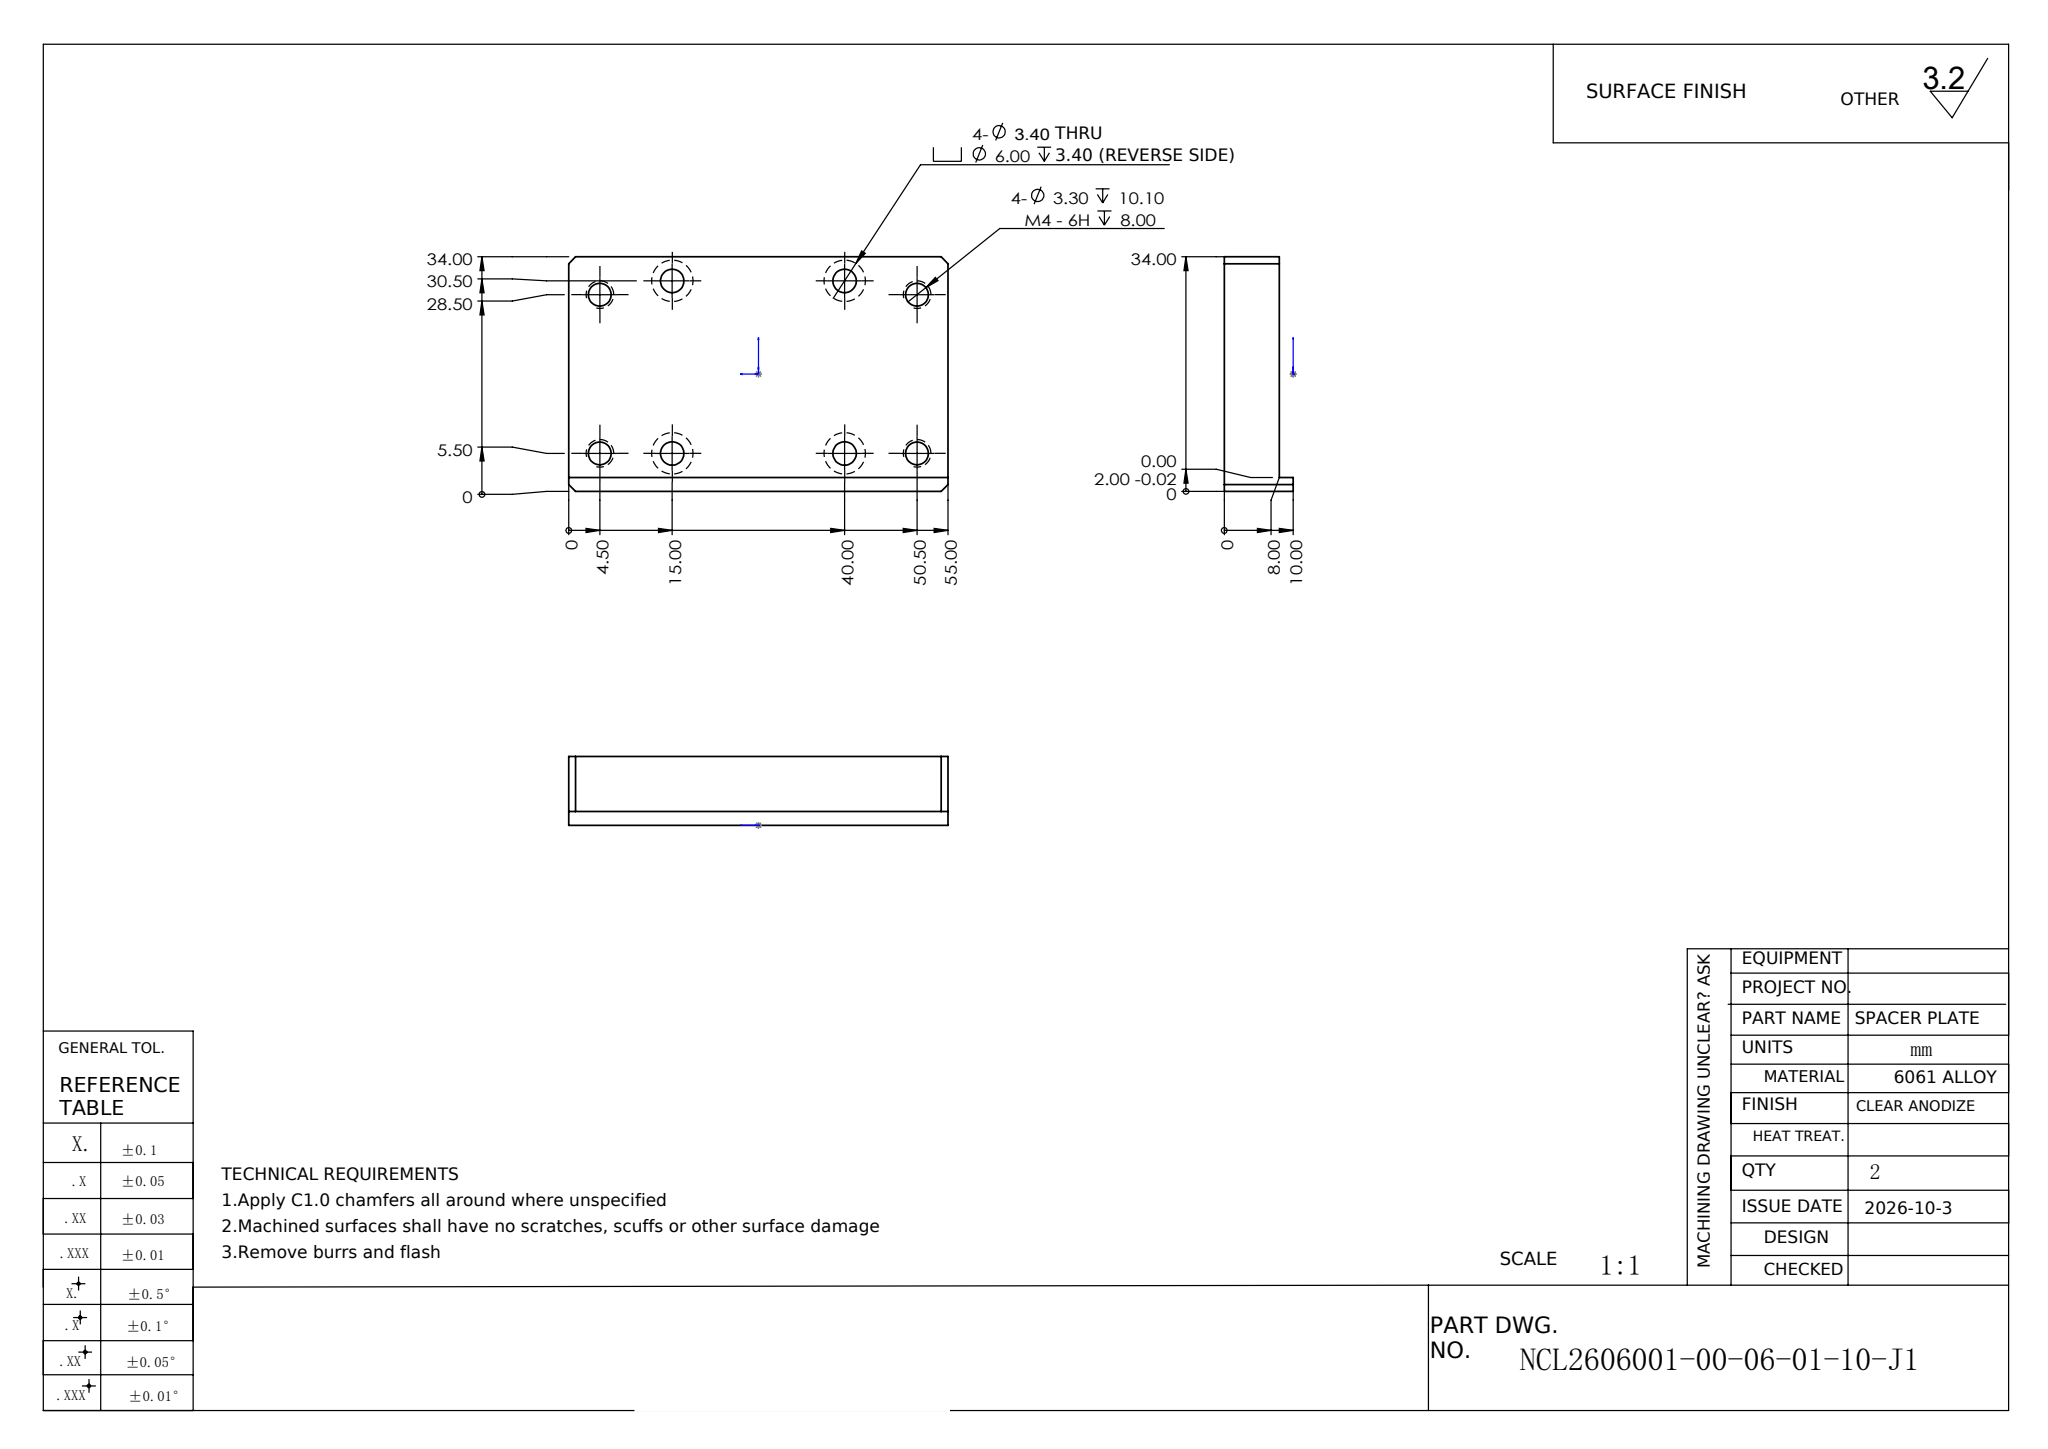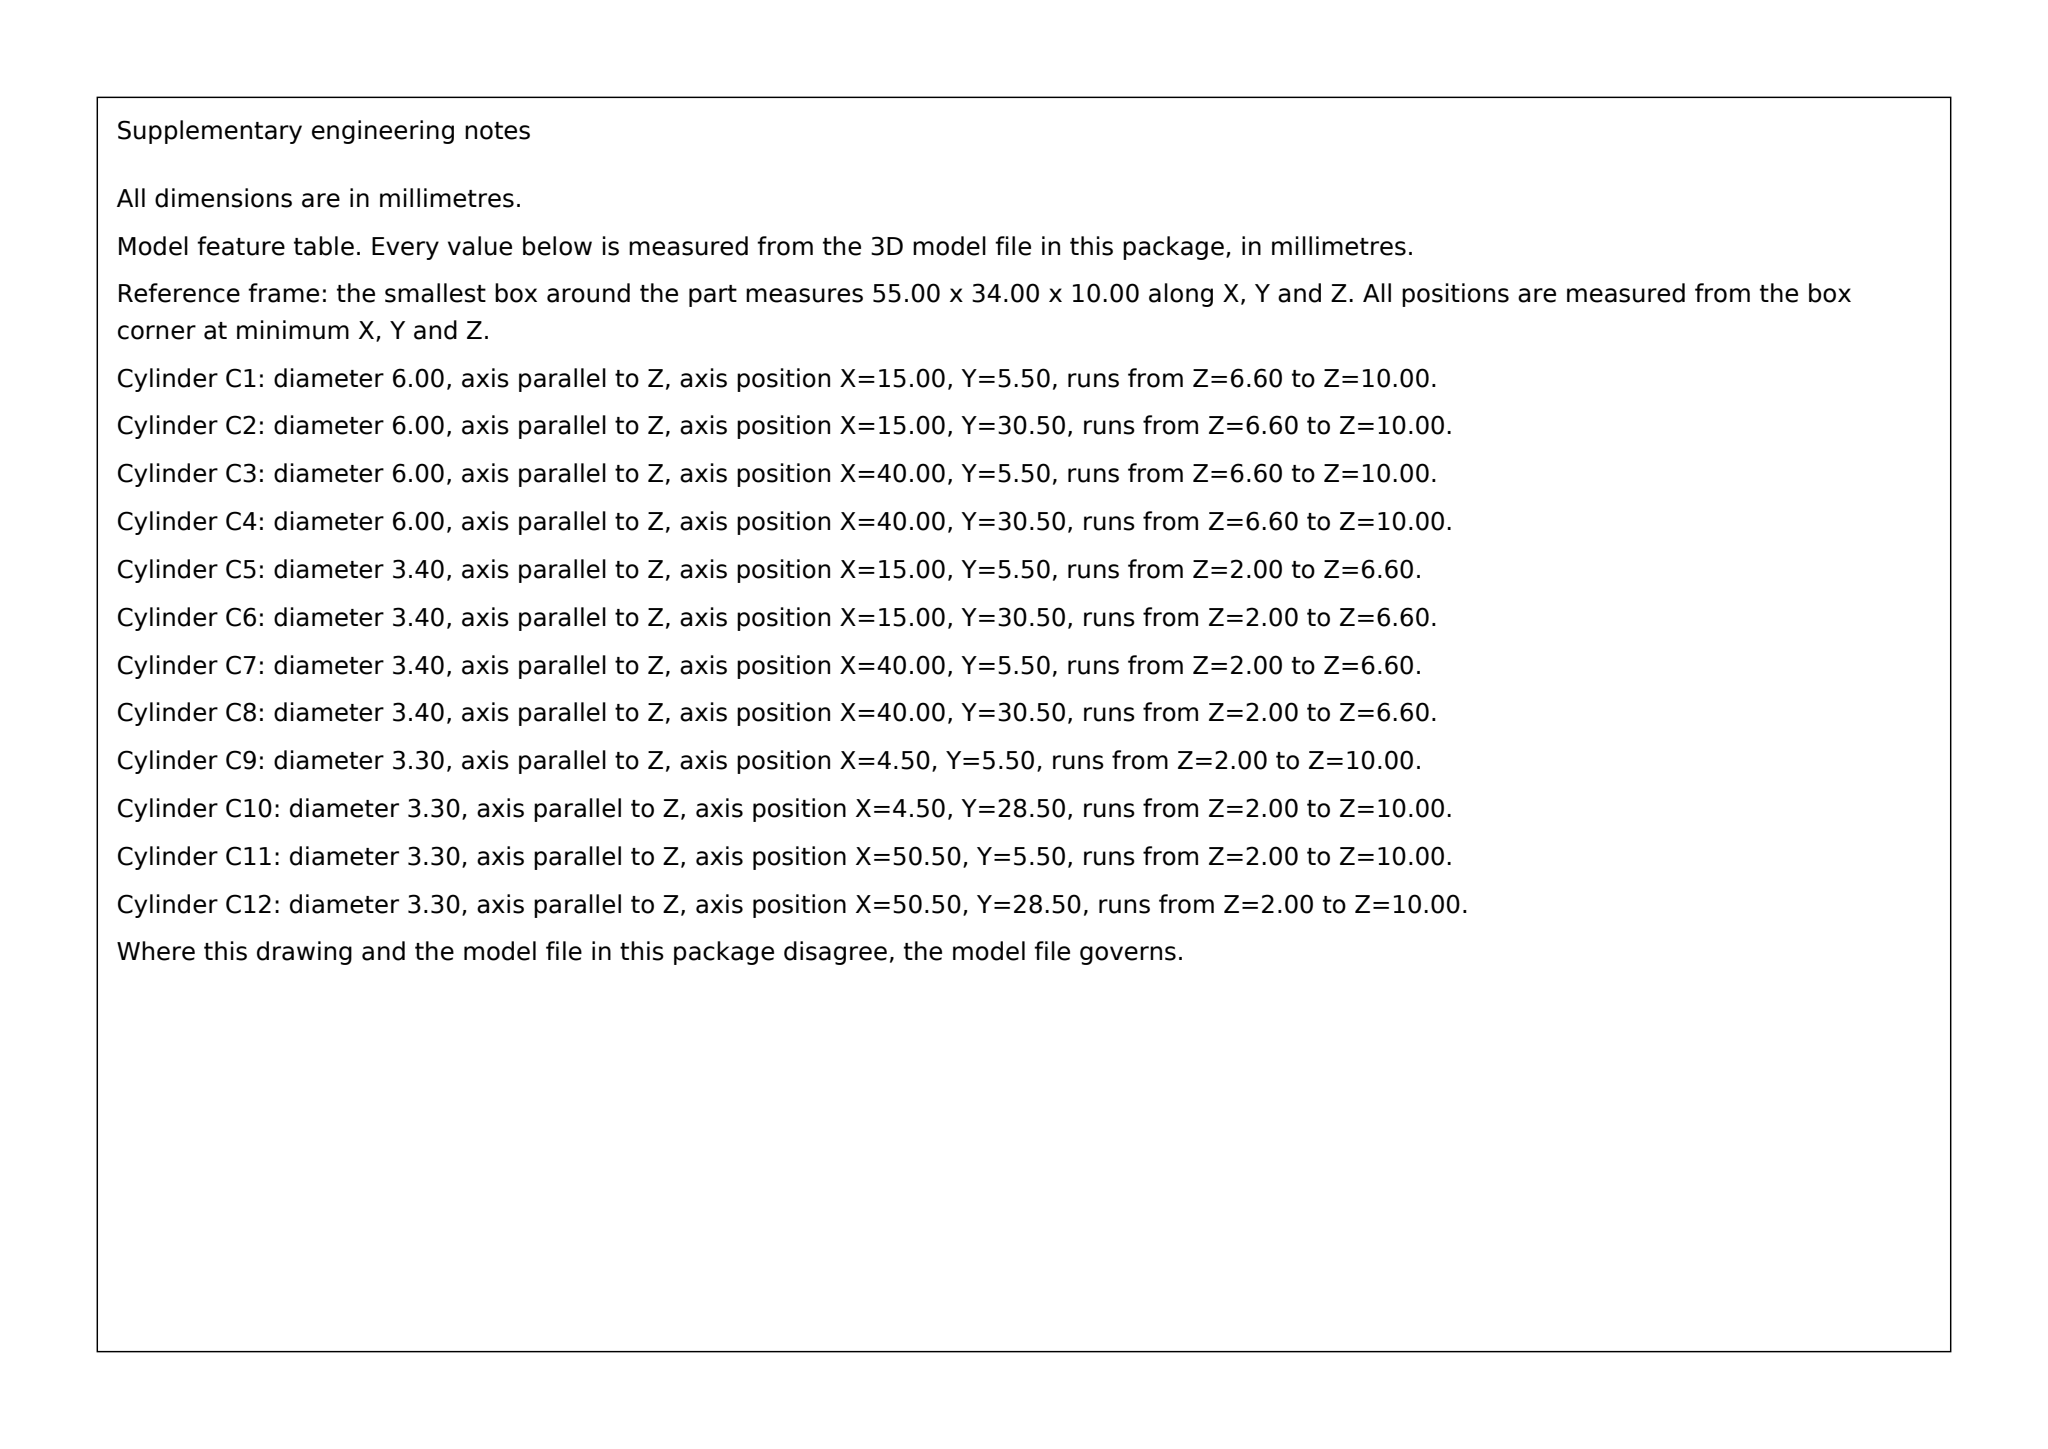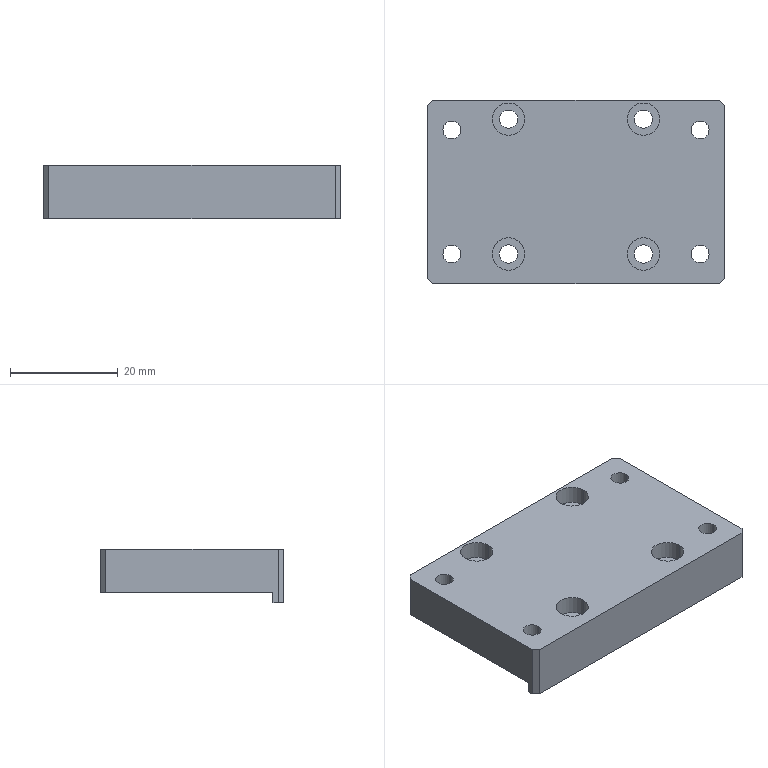Part | SolidWorks | mm | 1 solid | 40 faces | box 55 x 34 x 10 mm | volume 14337 mm3 | cylinder 24 | plane 16 | commonest cylinder face diameters 3.3 x8 6 x8 3.4 x8